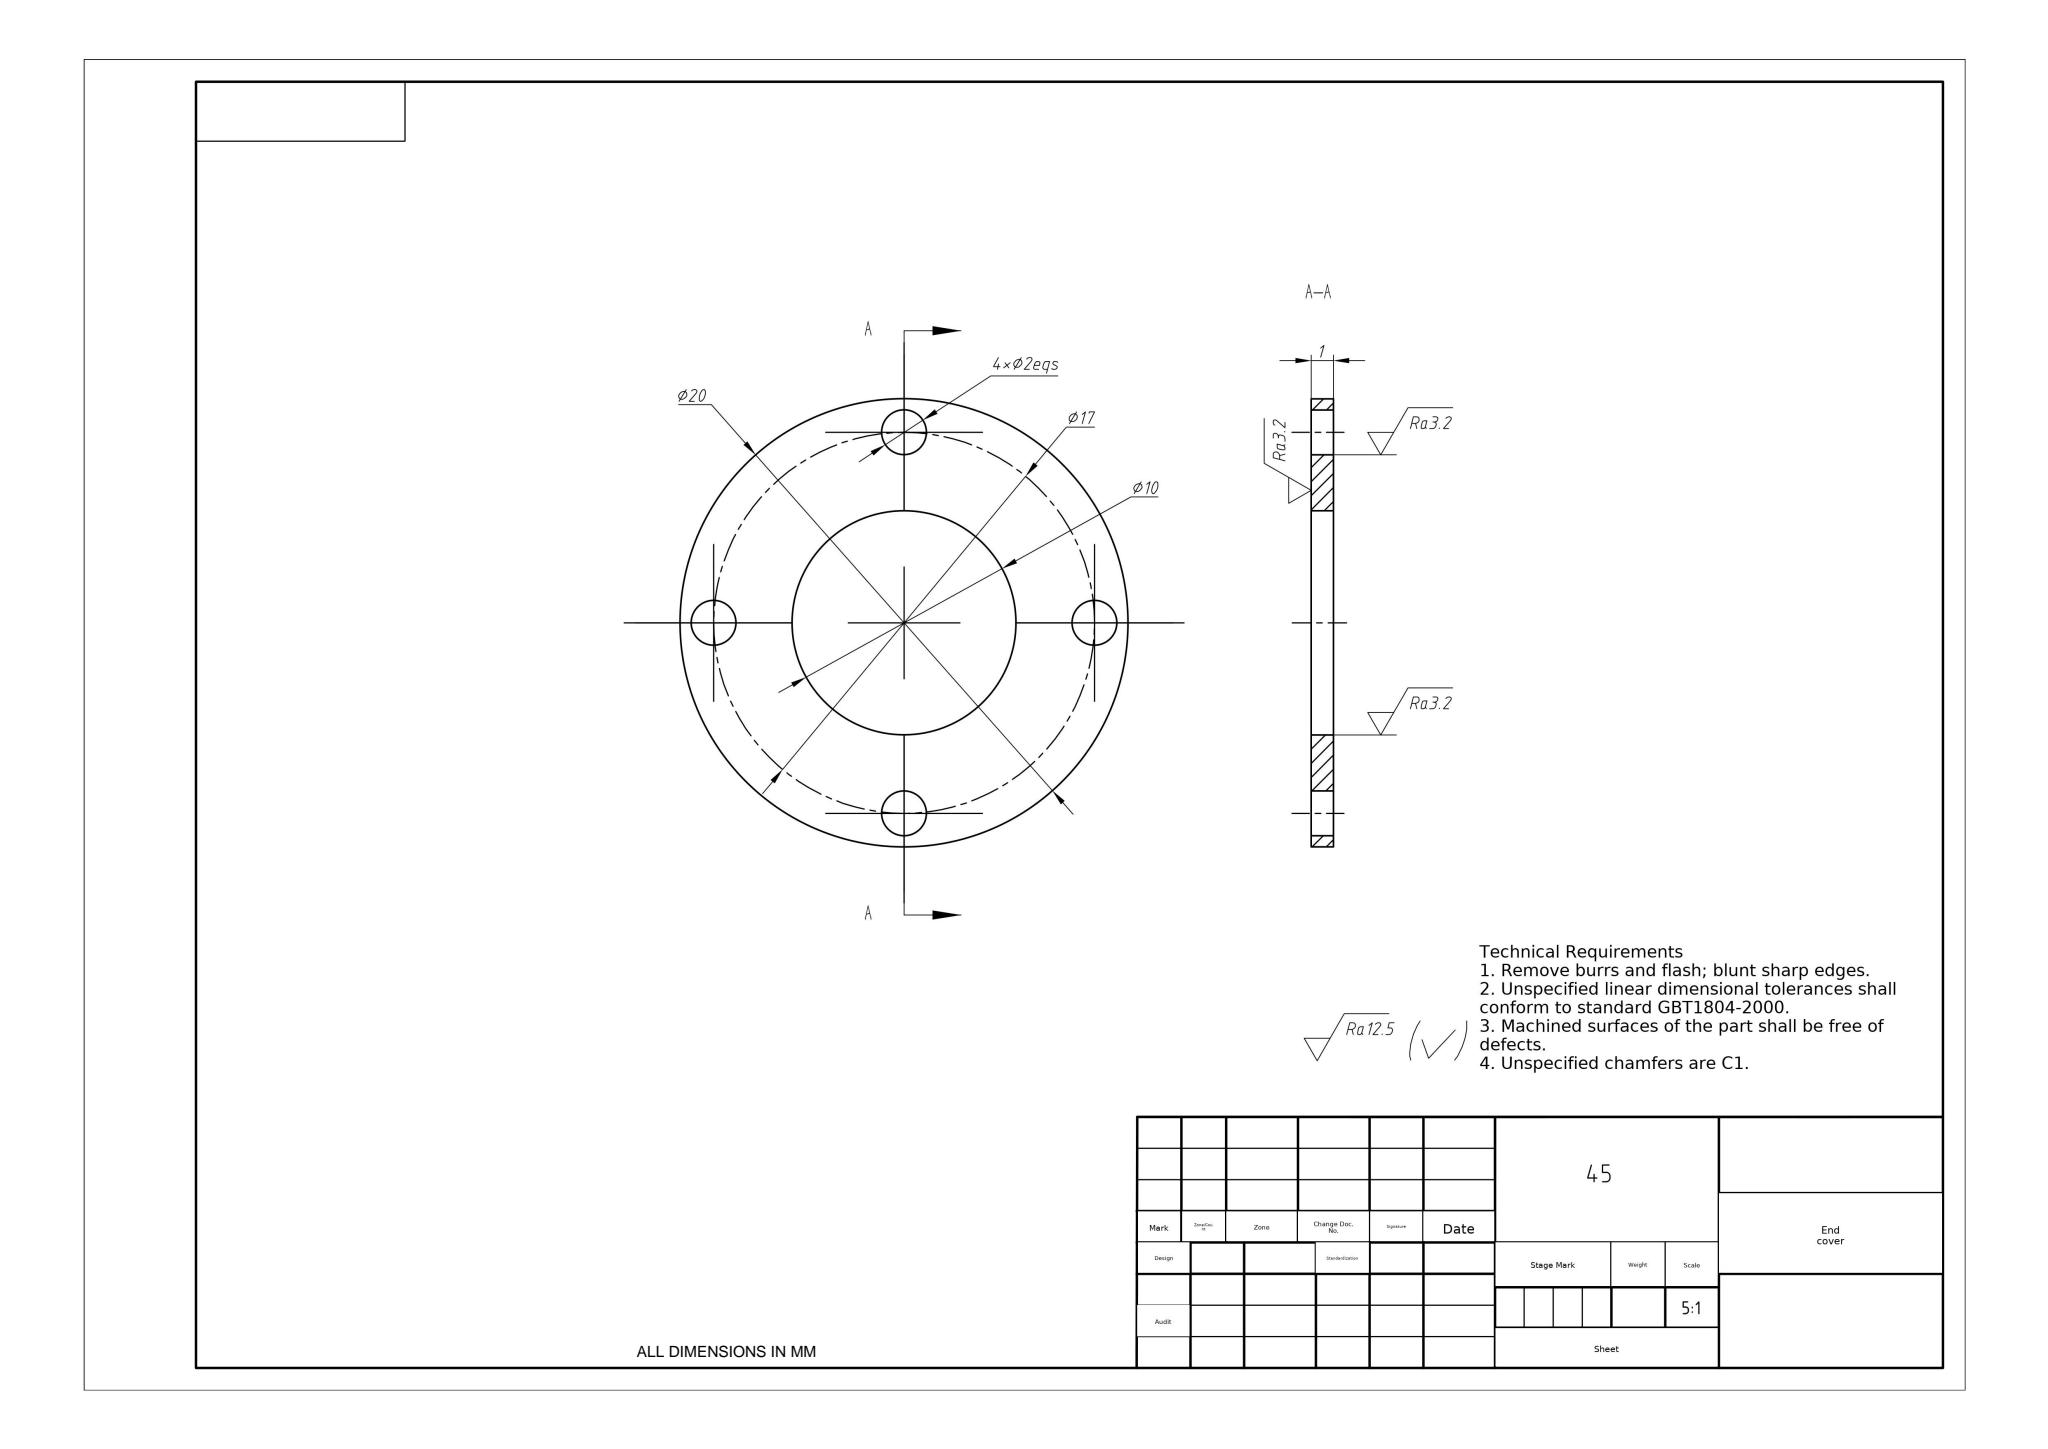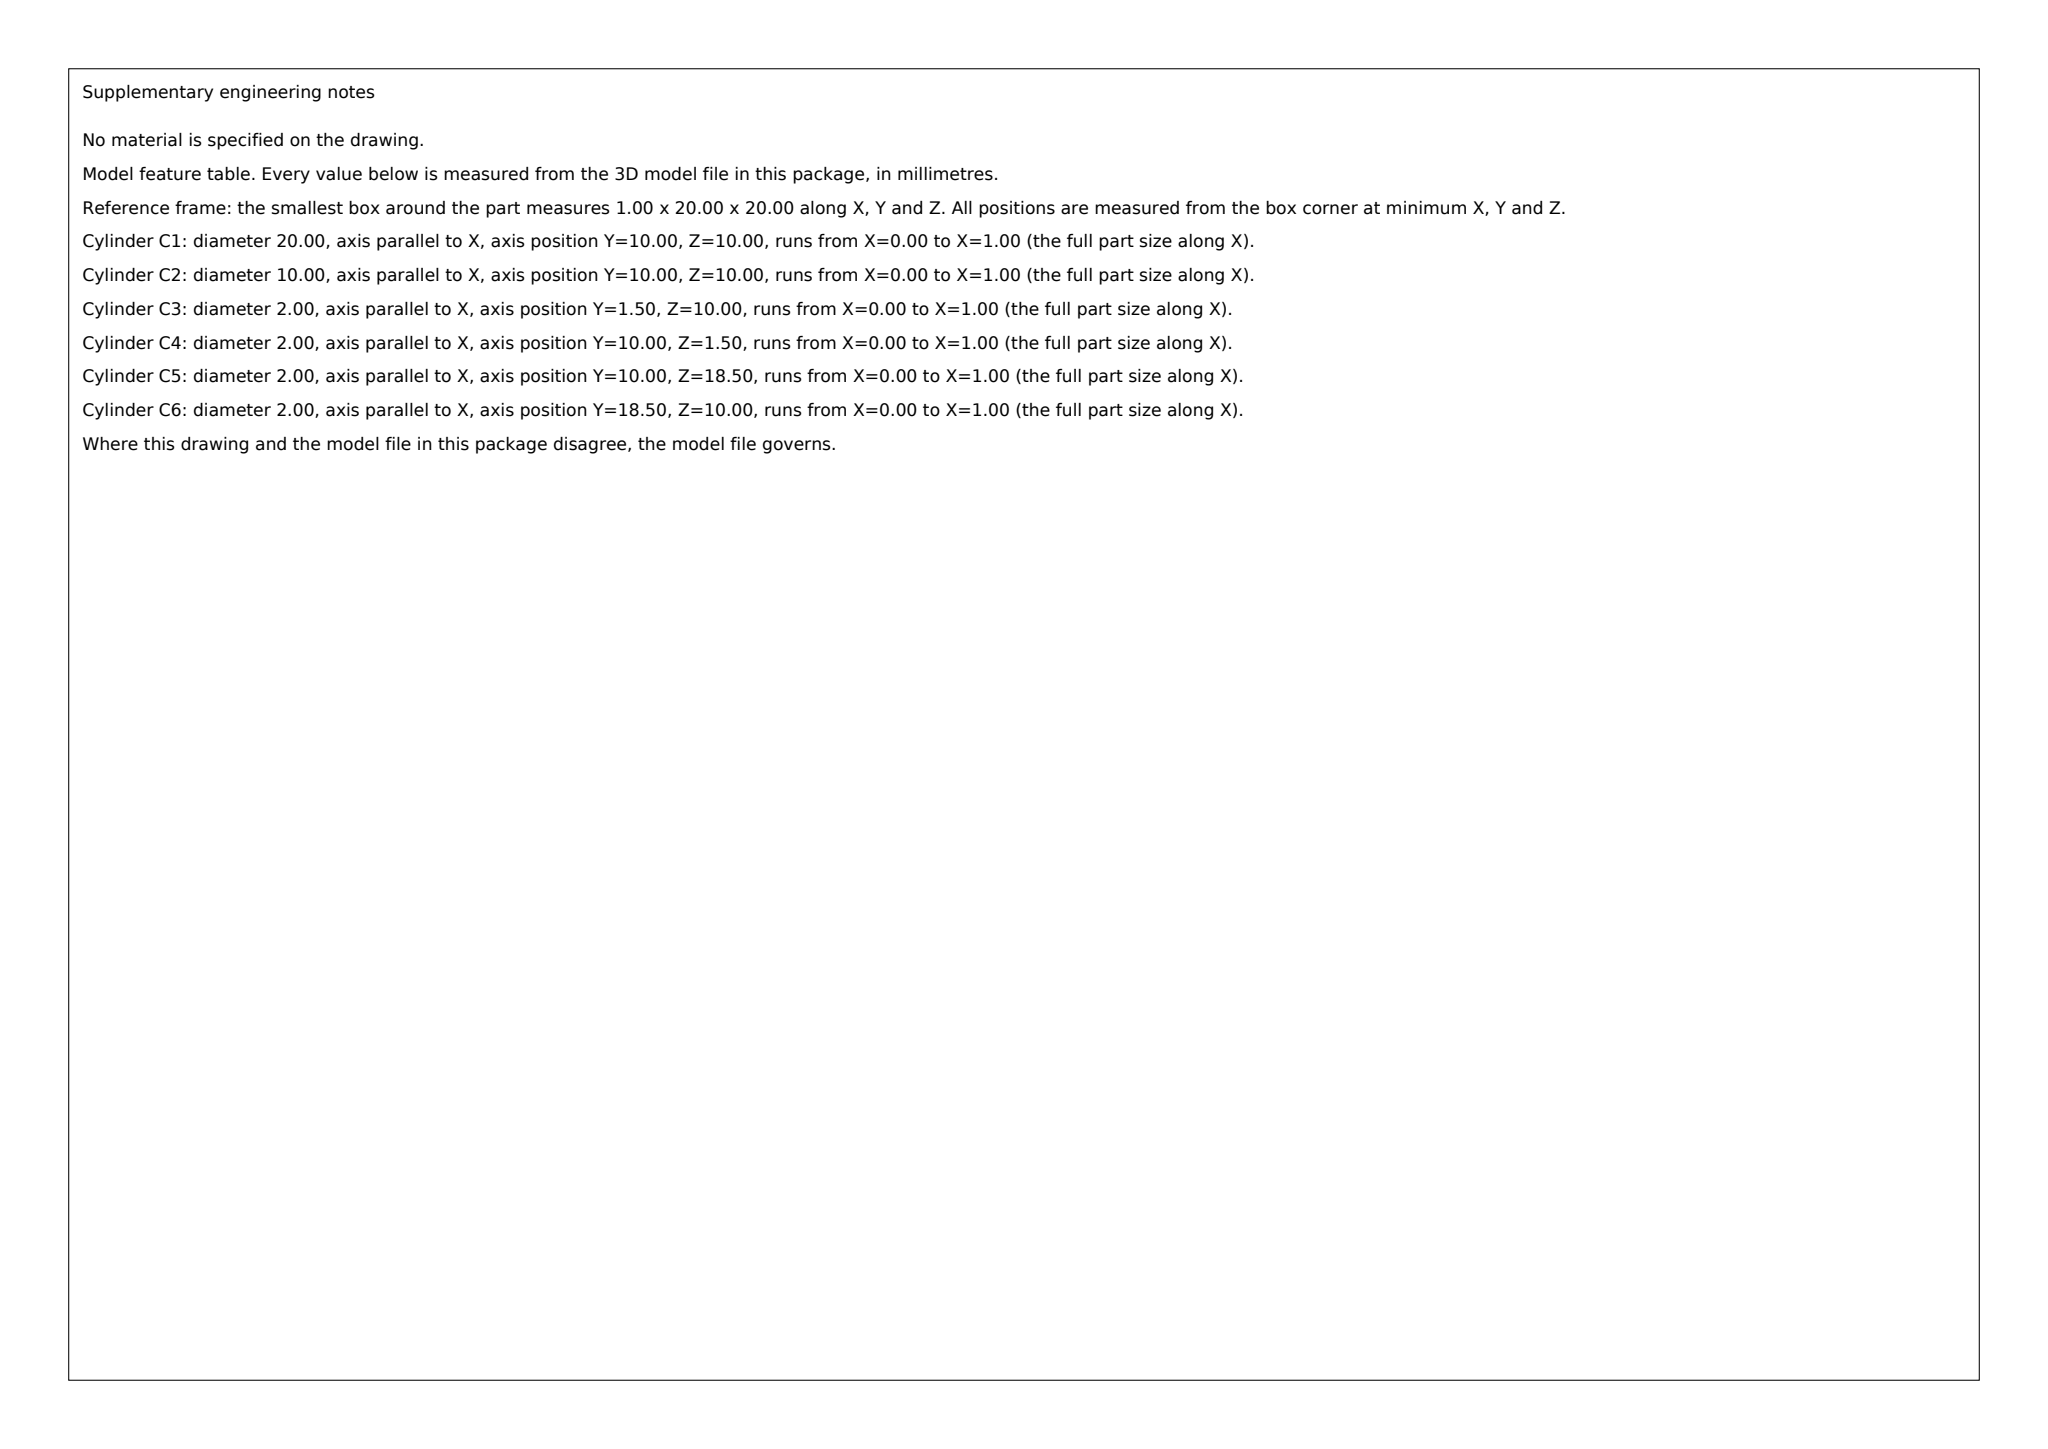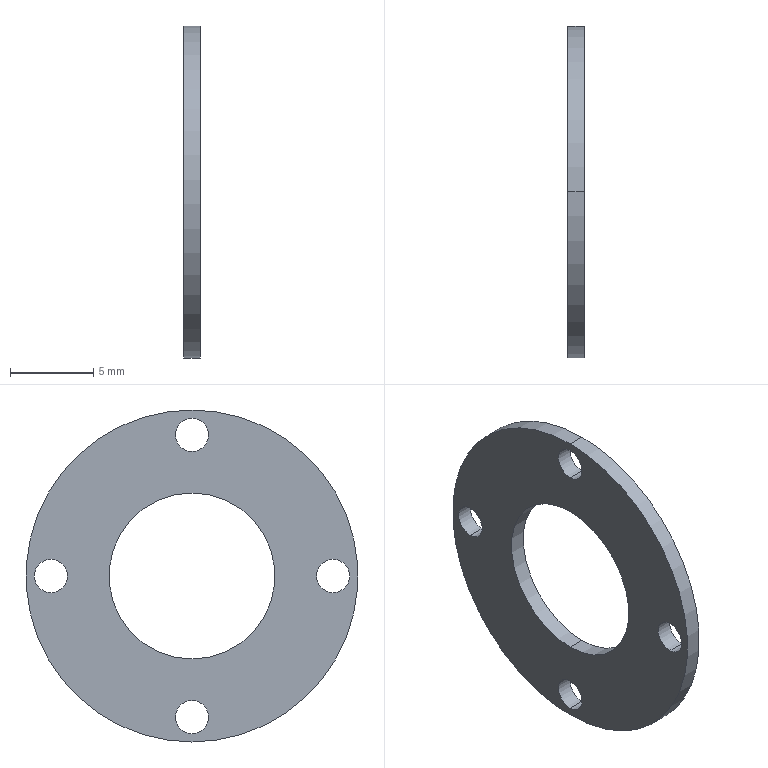Part | SolidWorks | mm | material 45 | 1 solid | 14 faces | box 1 x 20 x 20 mm | volume 223 mm3 | cylinder 12 | plane 2 | commonest cylinder face diameters 2 x8 10 x2 20 x2
build123d program:
from build123d import *

# Parameters (mm, degrees)
SKETCH1_R           = 10
SKETCH1_R_2         = 5
SKETCH1_R_3         = 1
BOSS_EXTRUDE1_DEPTH = 1


with BuildPart() as part:
    # Sketch1 → Boss-Extrude1 (new body)
    with BuildSketch(Plane(origin=(0, 0, 0), x_dir=(0, 0, -1), z_dir=(1, 0, 0))):
        Circle(SKETCH1_R)
        Circle(SKETCH1_R_2, mode=Mode.SUBTRACT)
        with Locations((0, 8.5)):
            Circle(SKETCH1_R_3, mode=Mode.SUBTRACT)
        with Locations((8.5, 0)):
            Circle(SKETCH1_R_3, mode=Mode.SUBTRACT)
        with Locations((0, -8.5)):
            Circle(SKETCH1_R_3, mode=Mode.SUBTRACT)
        with Locations((-8.5, 0)):
            Circle(SKETCH1_R_3, mode=Mode.SUBTRACT)
    extrude(amount=BOSS_EXTRUDE1_DEPTH)


solid = part.part
STEP:
#1=CARTESIAN_POINT('',(1.,0.,9.5));
#2=VERTEX_POINT('',#1);
#3=CARTESIAN_POINT('',(1.,0.,7.5));
#4=VERTEX_POINT('',#3);
#5=CARTESIAN_POINT('',(1.,0.,8.5));
#6=DIRECTION('',(1.,-0.,-0.));
#7=DIRECTION('',(0.,-0.,-1.));
#8=AXIS2_PLACEMENT_3D('',#5,#6,#7);
#9=CIRCLE('',#8,1.);
#10=EDGE_CURVE('',#2,#4,#9,.T.);
#11=ORIENTED_EDGE('',*,*,#10,.T.);
#12=CARTESIAN_POINT('',(-0.,0.,7.5));
#13=VERTEX_POINT('',#12);
#14=CARTESIAN_POINT('',(1.,0.,7.5));
#15=DIRECTION('',(-1.,0.,0.));
#16=VECTOR('',#15,1000.);
#17=LINE('',#14,#16);
#18=EDGE_CURVE('',#4,#13,#17,.T.);
#19=ORIENTED_EDGE('',*,*,#18,.T.);
#20=CARTESIAN_POINT('',(0.,0.,9.5));
#21=VERTEX_POINT('',#20);
#22=CARTESIAN_POINT('',(0.,0.,8.5));
#23=DIRECTION('',(1.,-0.,-0.));
#24=DIRECTION('',(0.,-0.,-1.));
#25=AXIS2_PLACEMENT_3D('',#22,#23,#24);
#26=CIRCLE('',#25,1.);
#27=EDGE_CURVE('',#21,#13,#26,.T.);
#28=ORIENTED_EDGE('',*,*,#27,.F.);
#29=CARTESIAN_POINT('',(1.,0.,9.5));
#30=DIRECTION('',(-1.,0.,0.));
#31=VECTOR('',#30,1000.);
#32=LINE('',#29,#31);
#33=EDGE_CURVE('',#2,#21,#32,.T.);
#34=ORIENTED_EDGE('',*,*,#33,.F.);
#35=EDGE_LOOP('',(#11,#19,#28,#34));
#36=FACE_OUTER_BOUND('',#35,.T.);
#37=CARTESIAN_POINT('',(1.,0.,8.5));
#38=DIRECTION('',(-1.,0.,0.));
#39=DIRECTION('',(-0.,0.,1.));
#40=AXIS2_PLACEMENT_3D('',#37,#38,#39);
#41=CYLINDRICAL_SURFACE('',#40,1.);
#42=ADVANCED_FACE('',(#36),#41,.F.);
#43=CARTESIAN_POINT('',(1.,-8.5,1.));
#44=VERTEX_POINT('',#43);
#45=CARTESIAN_POINT('',(1.,-8.5,-1.));
#46=VERTEX_POINT('',#45);
#47=CARTESIAN_POINT('',(1.,-8.5,0.));
#48=DIRECTION('',(1.,-0.,-0.));
#49=DIRECTION('',(0.,-0.,-1.));
#50=AXIS2_PLACEMENT_3D('',#47,#48,#49);
#51=CIRCLE('',#50,1.);
#52=EDGE_CURVE('',#44,#46,#51,.T.);
#53=ORIENTED_EDGE('',*,*,#52,.T.);
#54=CARTESIAN_POINT('',(-0.,-8.5,-1.));
#55=VERTEX_POINT('',#54);
#56=CARTESIAN_POINT('',(1.,-8.5,-1.));
#57=DIRECTION('',(-1.,0.,0.));
#58=VECTOR('',#57,1000.);
#59=LINE('',#56,#58);
#60=EDGE_CURVE('',#46,#55,#59,.T.);
#61=ORIENTED_EDGE('',*,*,#60,.T.);
#62=CARTESIAN_POINT('',(0.,-8.5,1.));
#63=VERTEX_POINT('',#62);
#64=CARTESIAN_POINT('',(0.,-8.5,0.));
#65=DIRECTION('',(1.,-0.,-0.));
#66=DIRECTION('',(0.,-0.,-1.));
#67=AXIS2_PLACEMENT_3D('',#64,#65,#66);
#68=CIRCLE('',#67,1.);
#69=EDGE_CURVE('',#63,#55,#68,.T.);
#70=ORIENTED_EDGE('',*,*,#69,.F.);
#71=CARTESIAN_POINT('',(1.,-8.5,1.));
#72=DIRECTION('',(-1.,0.,0.));
#73=VECTOR('',#72,1000.);
#74=LINE('',#71,#73);
#75=EDGE_CURVE('',#44,#63,#74,.T.);
#76=ORIENTED_EDGE('',*,*,#75,.F.);
#77=EDGE_LOOP('',(#53,#61,#70,#76));
#78=FACE_OUTER_BOUND('',#77,.T.);
#79=CARTESIAN_POINT('',(1.,-8.5,0.));
#80=DIRECTION('',(-1.,0.,0.));
#81=DIRECTION('',(-0.,0.,1.));
#82=AXIS2_PLACEMENT_3D('',#79,#80,#81);
#83=CYLINDRICAL_SURFACE('',#82,1.);
#84=ADVANCED_FACE('',(#78),#83,.F.);
#85=CARTESIAN_POINT('',(1.,-0.,-7.5));
#86=VERTEX_POINT('',#85);
#87=CARTESIAN_POINT('',(1.,-0.,-9.5));
#88=VERTEX_POINT('',#87);
#89=CARTESIAN_POINT('',(1.,-0.,-8.5));
#90=DIRECTION('',(1.,-0.,-0.));
#91=DIRECTION('',(0.,-0.,-1.));
#92=AXIS2_PLACEMENT_3D('',#89,#90,#91);
#93=CIRCLE('',#92,1.);
#94=EDGE_CURVE('',#86,#88,#93,.T.);
#95=ORIENTED_EDGE('',*,*,#94,.T.);
#96=CARTESIAN_POINT('',(-0.,-0.,-9.5));
#97=VERTEX_POINT('',#96);
#98=CARTESIAN_POINT('',(1.,-0.,-9.5));
#99=DIRECTION('',(-1.,0.,0.));
#100=VECTOR('',#99,1000.);
#101=LINE('',#98,#100);
#102=EDGE_CURVE('',#88,#97,#101,.T.);
#103=ORIENTED_EDGE('',*,*,#102,.T.);
#104=CARTESIAN_POINT('',(-0.,-0.,-7.5));
#105=VERTEX_POINT('',#104);
#106=CARTESIAN_POINT('',(-0.,-0.,-8.5));
#107=DIRECTION('',(1.,-0.,-0.));
#108=DIRECTION('',(0.,-0.,-1.));
#109=AXIS2_PLACEMENT_3D('',#106,#107,#108);
#110=CIRCLE('',#109,1.);
#111=EDGE_CURVE('',#105,#97,#110,.T.);
#112=ORIENTED_EDGE('',*,*,#111,.F.);
#113=CARTESIAN_POINT('',(1.,-0.,-7.5));
#114=DIRECTION('',(-1.,0.,0.));
#115=VECTOR('',#114,1000.);
#116=LINE('',#113,#115);
#117=EDGE_CURVE('',#86,#105,#116,.T.);
#118=ORIENTED_EDGE('',*,*,#117,.F.);
#119=EDGE_LOOP('',(#95,#103,#112,#118));
#120=FACE_OUTER_BOUND('',#119,.T.);
#121=CARTESIAN_POINT('',(1.,-0.,-8.5));
#122=DIRECTION('',(-1.,0.,0.));
#123=DIRECTION('',(-0.,0.,1.));
#124=AXIS2_PLACEMENT_3D('',#121,#122,#123);
#125=CYLINDRICAL_SURFACE('',#124,1.);
#126=ADVANCED_FACE('',(#120),#125,.F.);
#127=CARTESIAN_POINT('',(1.,8.5,1.));
#128=VERTEX_POINT('',#127);
#129=CARTESIAN_POINT('',(1.,8.5,-1.));
#130=VERTEX_POINT('',#129);
#131=CARTESIAN_POINT('',(1.,8.5,0.));
#132=DIRECTION('',(1.,-0.,-0.));
#133=DIRECTION('',(0.,-0.,-1.));
#134=AXIS2_PLACEMENT_3D('',#131,#132,#133);
#135=CIRCLE('',#134,1.);
#136=EDGE_CURVE('',#128,#130,#135,.T.);
#137=ORIENTED_EDGE('',*,*,#136,.T.);
#138=CARTESIAN_POINT('',(0.,8.5,-1.));
#139=VERTEX_POINT('',#138);
#140=CARTESIAN_POINT('',(1.,8.5,-1.));
#141=DIRECTION('',(-1.,0.,0.));
#142=VECTOR('',#141,1000.);
#143=LINE('',#140,#142);
#144=EDGE_CURVE('',#130,#139,#143,.T.);
#145=ORIENTED_EDGE('',*,*,#144,.T.);
#146=CARTESIAN_POINT('',(0.,8.5,1.));
#147=VERTEX_POINT('',#146);
#148=CARTESIAN_POINT('',(0.,8.5,0.));
#149=DIRECTION('',(1.,-0.,-0.));
#150=DIRECTION('',(0.,-0.,-1.));
#151=AXIS2_PLACEMENT_3D('',#148,#149,#150);
#152=CIRCLE('',#151,1.);
#153=EDGE_CURVE('',#147,#139,#152,.T.);
#154=ORIENTED_EDGE('',*,*,#153,.F.);
#155=CARTESIAN_POINT('',(1.,8.5,1.));
#156=DIRECTION('',(-1.,0.,0.));
#157=VECTOR('',#156,1000.);
#158=LINE('',#155,#157);
#159=EDGE_CURVE('',#128,#147,#158,.T.);
#160=ORIENTED_EDGE('',*,*,#159,.F.);
#161=EDGE_LOOP('',(#137,#145,#154,#160));
#162=FACE_OUTER_BOUND('',#161,.T.);
#163=CARTESIAN_POINT('',(1.,8.5,0.));
#164=DIRECTION('',(-1.,0.,0.));
#165=DIRECTION('',(-0.,0.,1.));
#166=AXIS2_PLACEMENT_3D('',#163,#164,#165);
#167=CYLINDRICAL_SURFACE('',#166,1.);
#168=ADVANCED_FACE('',(#162),#167,.F.);
#169=CARTESIAN_POINT('',(1.,0.,5.));
#170=VERTEX_POINT('',#169);
#171=CARTESIAN_POINT('',(1.,0.,-5.));
#172=VERTEX_POINT('',#171);
#173=CARTESIAN_POINT('',(1.,0.,0.));
#174=DIRECTION('',(1.,-0.,-0.));
#175=DIRECTION('',(0.,-0.,-1.));
#176=AXIS2_PLACEMENT_3D('',#173,#174,#175);
#177=CIRCLE('',#176,5.);
#178=EDGE_CURVE('',#170,#172,#177,.T.);
#179=ORIENTED_EDGE('',*,*,#178,.T.);
#180=CARTESIAN_POINT('',(-0.,0.,-5.));
#181=VERTEX_POINT('',#180);
#182=CARTESIAN_POINT('',(1.,0.,-5.));
#183=DIRECTION('',(-1.,0.,0.));
#184=VECTOR('',#183,1000.);
#185=LINE('',#182,#184);
#186=EDGE_CURVE('',#172,#181,#185,.T.);
#187=ORIENTED_EDGE('',*,*,#186,.T.);
#188=CARTESIAN_POINT('',(0.,0.,5.));
#189=VERTEX_POINT('',#188);
#190=CARTESIAN_POINT('',(0.,0.,0.));
#191=DIRECTION('',(1.,-0.,-0.));
#192=DIRECTION('',(0.,-0.,-1.));
#193=AXIS2_PLACEMENT_3D('',#190,#191,#192);
#194=CIRCLE('',#193,5.);
#195=EDGE_CURVE('',#189,#181,#194,.T.);
#196=ORIENTED_EDGE('',*,*,#195,.F.);
#197=CARTESIAN_POINT('',(1.,0.,5.));
#198=DIRECTION('',(-1.,0.,0.));
#199=VECTOR('',#198,1000.);
#200=LINE('',#197,#199);
#201=EDGE_CURVE('',#170,#189,#200,.T.);
#202=ORIENTED_EDGE('',*,*,#201,.F.);
#203=EDGE_LOOP('',(#179,#187,#196,#202));
#204=FACE_OUTER_BOUND('',#203,.T.);
#205=CARTESIAN_POINT('',(1.,0.,0.));
#206=DIRECTION('',(-1.,0.,0.));
#207=DIRECTION('',(-0.,0.,1.));
#208=AXIS2_PLACEMENT_3D('',#205,#206,#207);
#209=CYLINDRICAL_SURFACE('',#208,5.);
#210=ADVANCED_FACE('',(#204),#209,.F.);
#211=CARTESIAN_POINT('',(1.,0.,-10.));
#212=VERTEX_POINT('',#211);
#213=CARTESIAN_POINT('',(1.,0.,10.));
#214=VERTEX_POINT('',#213);
#215=CARTESIAN_POINT('',(1.,0.,0.));
#216=DIRECTION('',(1.,-0.,-0.));
#217=DIRECTION('',(0.,-0.,-1.));
#218=AXIS2_PLACEMENT_3D('',#215,#216,#217);
#219=CIRCLE('',#218,10.);
#220=EDGE_CURVE('',#212,#214,#219,.T.);
#221=ORIENTED_EDGE('',*,*,#220,.F.);
#222=CARTESIAN_POINT('',(-0.,0.,-10.));
#223=VERTEX_POINT('',#222);
#224=CARTESIAN_POINT('',(1.,0.,-10.));
#225=DIRECTION('',(-1.,0.,0.));
#226=VECTOR('',#225,1000.);
#227=LINE('',#224,#226);
#228=EDGE_CURVE('',#212,#223,#227,.T.);
#229=ORIENTED_EDGE('',*,*,#228,.T.);
#230=CARTESIAN_POINT('',(0.,0.,10.));
#231=VERTEX_POINT('',#230);
#232=CARTESIAN_POINT('',(0.,0.,0.));
#233=DIRECTION('',(1.,-0.,-0.));
#234=DIRECTION('',(0.,-0.,-1.));
#235=AXIS2_PLACEMENT_3D('',#232,#233,#234);
#236=CIRCLE('',#235,10.);
#237=EDGE_CURVE('',#223,#231,#236,.T.);
#238=ORIENTED_EDGE('',*,*,#237,.T.);
#239=CARTESIAN_POINT('',(1.,0.,10.));
#240=DIRECTION('',(-1.,0.,0.));
#241=VECTOR('',#240,1000.);
#242=LINE('',#239,#241);
#243=EDGE_CURVE('',#214,#231,#242,.T.);
#244=ORIENTED_EDGE('',*,*,#243,.F.);
#245=EDGE_LOOP('',(#221,#229,#238,#244));
#246=FACE_OUTER_BOUND('',#245,.T.);
#247=CARTESIAN_POINT('',(1.,0.,0.));
#248=DIRECTION('',(-1.,0.,0.));
#249=DIRECTION('',(-0.,0.,1.));
#250=AXIS2_PLACEMENT_3D('',#247,#248,#249);
#251=CYLINDRICAL_SURFACE('',#250,10.);
#252=ADVANCED_FACE('',(#246),#251,.T.);
#253=ORIENTED_EDGE('',*,*,#52,.F.);
#254=CARTESIAN_POINT('',(1.,-8.5,0.));
#255=DIRECTION('',(1.,-0.,-0.));
#256=DIRECTION('',(0.,-0.,-1.));
#257=AXIS2_PLACEMENT_3D('',#254,#255,#256);
#258=CIRCLE('',#257,1.);
#259=EDGE_CURVE('',#46,#44,#258,.T.);
#260=ORIENTED_EDGE('',*,*,#259,.F.);
#261=EDGE_LOOP('',(#253,#260));
#262=FACE_BOUND('',#261,.T.);
#263=ORIENTED_EDGE('',*,*,#136,.F.);
#264=CARTESIAN_POINT('',(1.,8.5,0.));
#265=DIRECTION('',(1.,-0.,-0.));
#266=DIRECTION('',(0.,-0.,-1.));
#267=AXIS2_PLACEMENT_3D('',#264,#265,#266);
#268=CIRCLE('',#267,1.);
#269=EDGE_CURVE('',#130,#128,#268,.T.);
#270=ORIENTED_EDGE('',*,*,#269,.F.);
#271=EDGE_LOOP('',(#263,#270));
#272=FACE_BOUND('',#271,.T.);
#273=CARTESIAN_POINT('',(1.,0.,0.));
#274=DIRECTION('',(1.,-0.,-0.));
#275=DIRECTION('',(0.,-0.,-1.));
#276=AXIS2_PLACEMENT_3D('',#273,#274,#275);
#277=CIRCLE('',#276,10.);
#278=EDGE_CURVE('',#214,#212,#277,.T.);
#279=ORIENTED_EDGE('',*,*,#278,.T.);
#280=ORIENTED_EDGE('',*,*,#220,.T.);
#281=EDGE_LOOP('',(#279,#280));
#282=FACE_OUTER_BOUND('',#281,.T.);
#283=ORIENTED_EDGE('',*,*,#178,.F.);
#284=CARTESIAN_POINT('',(1.,0.,0.));
#285=DIRECTION('',(1.,-0.,-0.));
#286=DIRECTION('',(0.,-0.,-1.));
#287=AXIS2_PLACEMENT_3D('',#284,#285,#286);
#288=CIRCLE('',#287,5.);
#289=EDGE_CURVE('',#172,#170,#288,.T.);
#290=ORIENTED_EDGE('',*,*,#289,.F.);
#291=EDGE_LOOP('',(#283,#290));
#292=FACE_BOUND('',#291,.T.);
#293=ORIENTED_EDGE('',*,*,#94,.F.);
#294=CARTESIAN_POINT('',(1.,-0.,-8.5));
#295=DIRECTION('',(1.,-0.,-0.));
#296=DIRECTION('',(0.,-0.,-1.));
#297=AXIS2_PLACEMENT_3D('',#294,#295,#296);
#298=CIRCLE('',#297,1.);
#299=EDGE_CURVE('',#88,#86,#298,.T.);
#300=ORIENTED_EDGE('',*,*,#299,.F.);
#301=EDGE_LOOP('',(#293,#300));
#302=FACE_BOUND('',#301,.T.);
#303=ORIENTED_EDGE('',*,*,#10,.F.);
#304=CARTESIAN_POINT('',(1.,0.,8.5));
#305=DIRECTION('',(1.,-0.,-0.));
#306=DIRECTION('',(0.,-0.,-1.));
#307=AXIS2_PLACEMENT_3D('',#304,#305,#306);
#308=CIRCLE('',#307,1.);
#309=EDGE_CURVE('',#4,#2,#308,.T.);
#310=ORIENTED_EDGE('',*,*,#309,.F.);
#311=EDGE_LOOP('',(#303,#310));
#312=FACE_BOUND('',#311,.T.);
#313=CARTESIAN_POINT('',(1.,0.,0.));
#314=DIRECTION('',(1.,-0.,0.));
#315=DIRECTION('',(0.,-0.,-1.));
#316=AXIS2_PLACEMENT_3D('',#313,#314,#315);
#317=PLANE('',#316);
#318=ADVANCED_FACE('',(#262,#272,#282,#292,#302,#312),#317,.T.);
#319=CARTESIAN_POINT('',(0.,0.,0.));
#320=DIRECTION('',(1.,-0.,-0.));
#321=DIRECTION('',(0.,-0.,-1.));
#322=AXIS2_PLACEMENT_3D('',#319,#320,#321);
#323=CIRCLE('',#322,10.);
#324=EDGE_CURVE('',#231,#223,#323,.T.);
#325=ORIENTED_EDGE('',*,*,#324,.F.);
#326=ORIENTED_EDGE('',*,*,#237,.F.);
#327=EDGE_LOOP('',(#325,#326));
#328=FACE_OUTER_BOUND('',#327,.T.);
#329=ORIENTED_EDGE('',*,*,#195,.T.);
#330=CARTESIAN_POINT('',(0.,0.,0.));
#331=DIRECTION('',(1.,-0.,-0.));
#332=DIRECTION('',(0.,-0.,-1.));
#333=AXIS2_PLACEMENT_3D('',#330,#331,#332);
#334=CIRCLE('',#333,5.);
#335=EDGE_CURVE('',#181,#189,#334,.T.);
#336=ORIENTED_EDGE('',*,*,#335,.T.);
#337=EDGE_LOOP('',(#329,#336));
#338=FACE_BOUND('',#337,.T.);
#339=ORIENTED_EDGE('',*,*,#153,.T.);
#340=CARTESIAN_POINT('',(0.,8.5,0.));
#341=DIRECTION('',(1.,-0.,-0.));
#342=DIRECTION('',(0.,-0.,-1.));
#343=AXIS2_PLACEMENT_3D('',#340,#341,#342);
#344=CIRCLE('',#343,1.);
#345=EDGE_CURVE('',#139,#147,#344,.T.);
#346=ORIENTED_EDGE('',*,*,#345,.T.);
#347=EDGE_LOOP('',(#339,#346));
#348=FACE_BOUND('',#347,.T.);
#349=ORIENTED_EDGE('',*,*,#111,.T.);
#350=CARTESIAN_POINT('',(-0.,-0.,-8.5));
#351=DIRECTION('',(1.,-0.,-0.));
#352=DIRECTION('',(0.,-0.,-1.));
#353=AXIS2_PLACEMENT_3D('',#350,#351,#352);
#354=CIRCLE('',#353,1.);
#355=EDGE_CURVE('',#97,#105,#354,.T.);
#356=ORIENTED_EDGE('',*,*,#355,.T.);
#357=EDGE_LOOP('',(#349,#356));
#358=FACE_BOUND('',#357,.T.);
#359=ORIENTED_EDGE('',*,*,#69,.T.);
#360=CARTESIAN_POINT('',(0.,-8.5,0.));
#361=DIRECTION('',(1.,-0.,-0.));
#362=DIRECTION('',(0.,-0.,-1.));
#363=AXIS2_PLACEMENT_3D('',#360,#361,#362);
#364=CIRCLE('',#363,1.);
#365=EDGE_CURVE('',#55,#63,#364,.T.);
#366=ORIENTED_EDGE('',*,*,#365,.T.);
#367=EDGE_LOOP('',(#359,#366));
#368=FACE_BOUND('',#367,.T.);
#369=ORIENTED_EDGE('',*,*,#27,.T.);
#370=CARTESIAN_POINT('',(0.,0.,8.5));
#371=DIRECTION('',(1.,-0.,-0.));
#372=DIRECTION('',(0.,-0.,-1.));
#373=AXIS2_PLACEMENT_3D('',#370,#371,#372);
#374=CIRCLE('',#373,1.);
#375=EDGE_CURVE('',#13,#21,#374,.T.);
#376=ORIENTED_EDGE('',*,*,#375,.T.);
#377=EDGE_LOOP('',(#369,#376));
#378=FACE_BOUND('',#377,.T.);
#379=CARTESIAN_POINT('',(0.,0.,0.));
#380=DIRECTION('',(1.,-0.,0.));
#381=DIRECTION('',(0.,-0.,-1.));
#382=AXIS2_PLACEMENT_3D('',#379,#380,#381);
#383=PLANE('',#382);
#384=ADVANCED_FACE('',(#328,#338,#348,#358,#368,#378),#383,.F.);
#385=ORIENTED_EDGE('',*,*,#228,.F.);
#386=ORIENTED_EDGE('',*,*,#278,.F.);
#387=ORIENTED_EDGE('',*,*,#243,.T.);
#388=ORIENTED_EDGE('',*,*,#324,.T.);
#389=EDGE_LOOP('',(#385,#386,#387,#388));
#390=FACE_OUTER_BOUND('',#389,.T.);
#391=CARTESIAN_POINT('',(1.,0.,0.));
#392=DIRECTION('',(-1.,0.,0.));
#393=DIRECTION('',(-0.,0.,1.));
#394=AXIS2_PLACEMENT_3D('',#391,#392,#393);
#395=CYLINDRICAL_SURFACE('',#394,10.);
#396=ADVANCED_FACE('',(#390),#395,.T.);
#397=ORIENTED_EDGE('',*,*,#186,.F.);
#398=ORIENTED_EDGE('',*,*,#289,.T.);
#399=ORIENTED_EDGE('',*,*,#201,.T.);
#400=ORIENTED_EDGE('',*,*,#335,.F.);
#401=EDGE_LOOP('',(#397,#398,#399,#400));
#402=FACE_OUTER_BOUND('',#401,.T.);
#403=CARTESIAN_POINT('',(1.,0.,0.));
#404=DIRECTION('',(-1.,0.,0.));
#405=DIRECTION('',(-0.,0.,1.));
#406=AXIS2_PLACEMENT_3D('',#403,#404,#405);
#407=CYLINDRICAL_SURFACE('',#406,5.);
#408=ADVANCED_FACE('',(#402),#407,.F.);
#409=ORIENTED_EDGE('',*,*,#144,.F.);
#410=ORIENTED_EDGE('',*,*,#269,.T.);
#411=ORIENTED_EDGE('',*,*,#159,.T.);
#412=ORIENTED_EDGE('',*,*,#345,.F.);
#413=EDGE_LOOP('',(#409,#410,#411,#412));
#414=FACE_OUTER_BOUND('',#413,.T.);
#415=CARTESIAN_POINT('',(1.,8.5,0.));
#416=DIRECTION('',(-1.,0.,0.));
#417=DIRECTION('',(-0.,0.,1.));
#418=AXIS2_PLACEMENT_3D('',#415,#416,#417);
#419=CYLINDRICAL_SURFACE('',#418,1.);
#420=ADVANCED_FACE('',(#414),#419,.F.);
#421=ORIENTED_EDGE('',*,*,#102,.F.);
#422=ORIENTED_EDGE('',*,*,#299,.T.);
#423=ORIENTED_EDGE('',*,*,#117,.T.);
#424=ORIENTED_EDGE('',*,*,#355,.F.);
#425=EDGE_LOOP('',(#421,#422,#423,#424));
#426=FACE_OUTER_BOUND('',#425,.T.);
#427=CARTESIAN_POINT('',(1.,-0.,-8.5));
#428=DIRECTION('',(-1.,0.,0.));
#429=DIRECTION('',(-0.,0.,1.));
#430=AXIS2_PLACEMENT_3D('',#427,#428,#429);
#431=CYLINDRICAL_SURFACE('',#430,1.);
#432=ADVANCED_FACE('',(#426),#431,.F.);
#433=ORIENTED_EDGE('',*,*,#60,.F.);
#434=ORIENTED_EDGE('',*,*,#259,.T.);
#435=ORIENTED_EDGE('',*,*,#75,.T.);
#436=ORIENTED_EDGE('',*,*,#365,.F.);
#437=EDGE_LOOP('',(#433,#434,#435,#436));
#438=FACE_OUTER_BOUND('',#437,.T.);
#439=CARTESIAN_POINT('',(1.,-8.5,0.));
#440=DIRECTION('',(-1.,0.,0.));
#441=DIRECTION('',(-0.,0.,1.));
#442=AXIS2_PLACEMENT_3D('',#439,#440,#441);
#443=CYLINDRICAL_SURFACE('',#442,1.);
#444=ADVANCED_FACE('',(#438),#443,.F.);
#445=ORIENTED_EDGE('',*,*,#18,.F.);
#446=ORIENTED_EDGE('',*,*,#309,.T.);
#447=ORIENTED_EDGE('',*,*,#33,.T.);
#448=ORIENTED_EDGE('',*,*,#375,.F.);
#449=EDGE_LOOP('',(#445,#446,#447,#448));
#450=FACE_OUTER_BOUND('',#449,.T.);
#451=CARTESIAN_POINT('',(1.,0.,8.5));
#452=DIRECTION('',(-1.,0.,0.));
#453=DIRECTION('',(-0.,0.,1.));
#454=AXIS2_PLACEMENT_3D('',#451,#452,#453);
#455=CYLINDRICAL_SURFACE('',#454,1.);
#456=ADVANCED_FACE('',(#450),#455,.F.);
#457=CLOSED_SHELL('',(#42,#84,#126,#168,#210,#252,#318,#384,#396,#408,#420,#432,#444,#456));
#458=MANIFOLD_SOLID_BREP('',#457);
#459=CARTESIAN_POINT('',(0.,0.,0.));
#460=DIRECTION('',(0.,0.,1.));
#461=DIRECTION('',(1.,0.,0.));
#462=AXIS2_PLACEMENT_3D('',#459,#460,#461);
#463=(LENGTH_UNIT()NAMED_UNIT(*)SI_UNIT(.MILLI.,.METRE.));
#464=UNCERTAINTY_MEASURE_WITH_UNIT(LENGTH_MEASURE(0.00001),#463,'','');
#465=(NAMED_UNIT(*)PLANE_ANGLE_UNIT()SI_UNIT($,.RADIAN.));
#466=(NAMED_UNIT(*)SI_UNIT($,.STERADIAN.)SOLID_ANGLE_UNIT());
#467=(GEOMETRIC_REPRESENTATION_CONTEXT(3)GLOBAL_UNCERTAINTY_ASSIGNED_CONTEXT((#464))GLOBAL_UNIT_ASSIGNED_CONTEXT((#463,#465,#466))REPRESENTATION_CONTEXT('',''));
#468=ADVANCED_BREP_SHAPE_REPRESENTATION('',(#458,#462),#467);